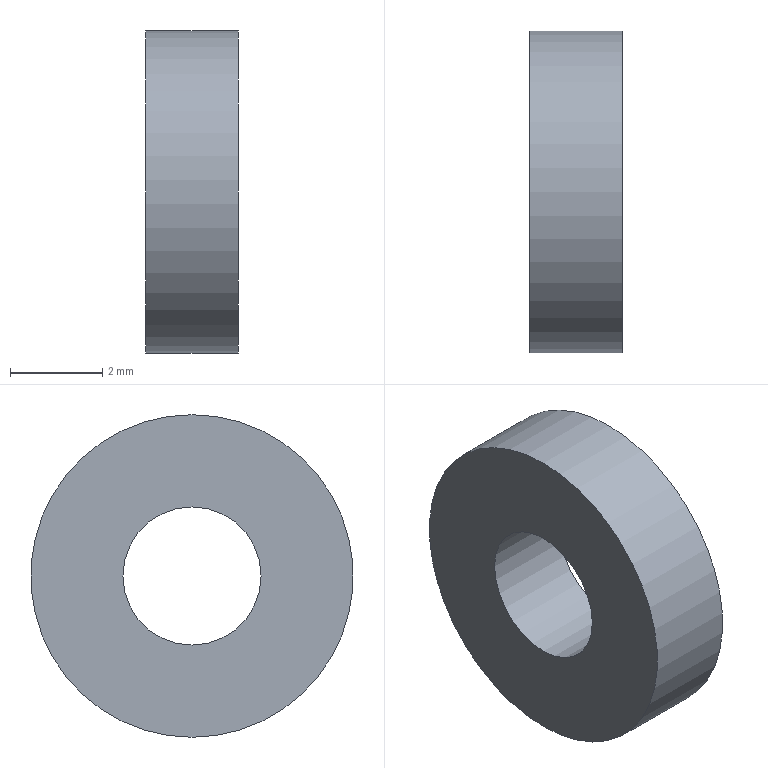Component | NX | EXT_CYLINDER_BODY_WASHER | 1 solid | 4 faces | volume 63 mm3 | cylinder 2 | plane 2 | commonest cylinder face diameters 7 x1 3 x1